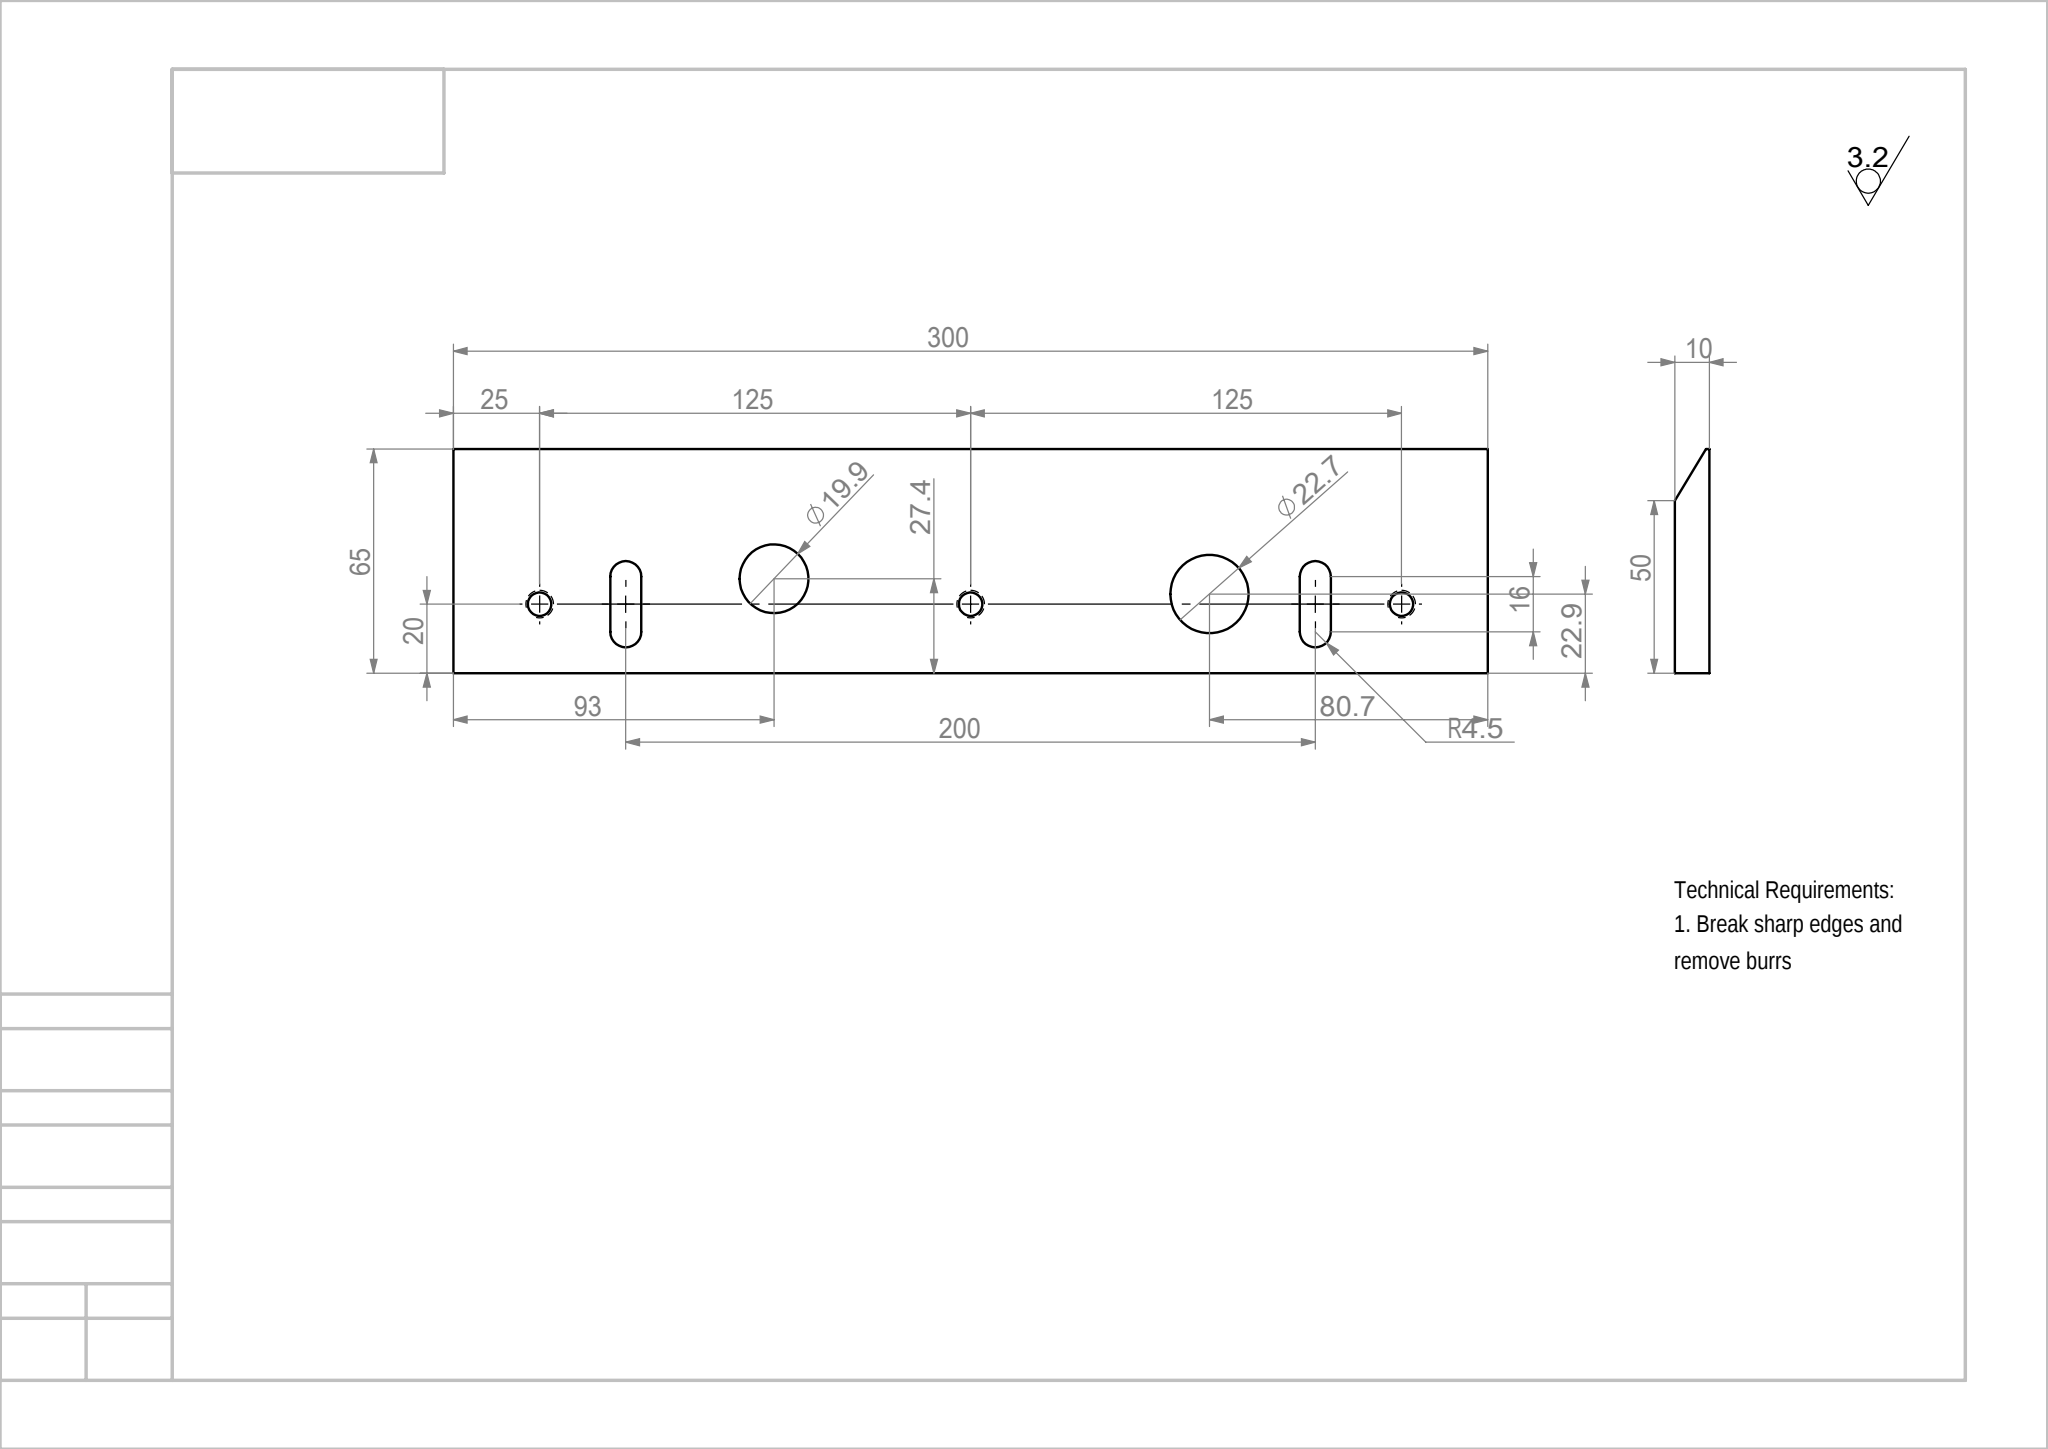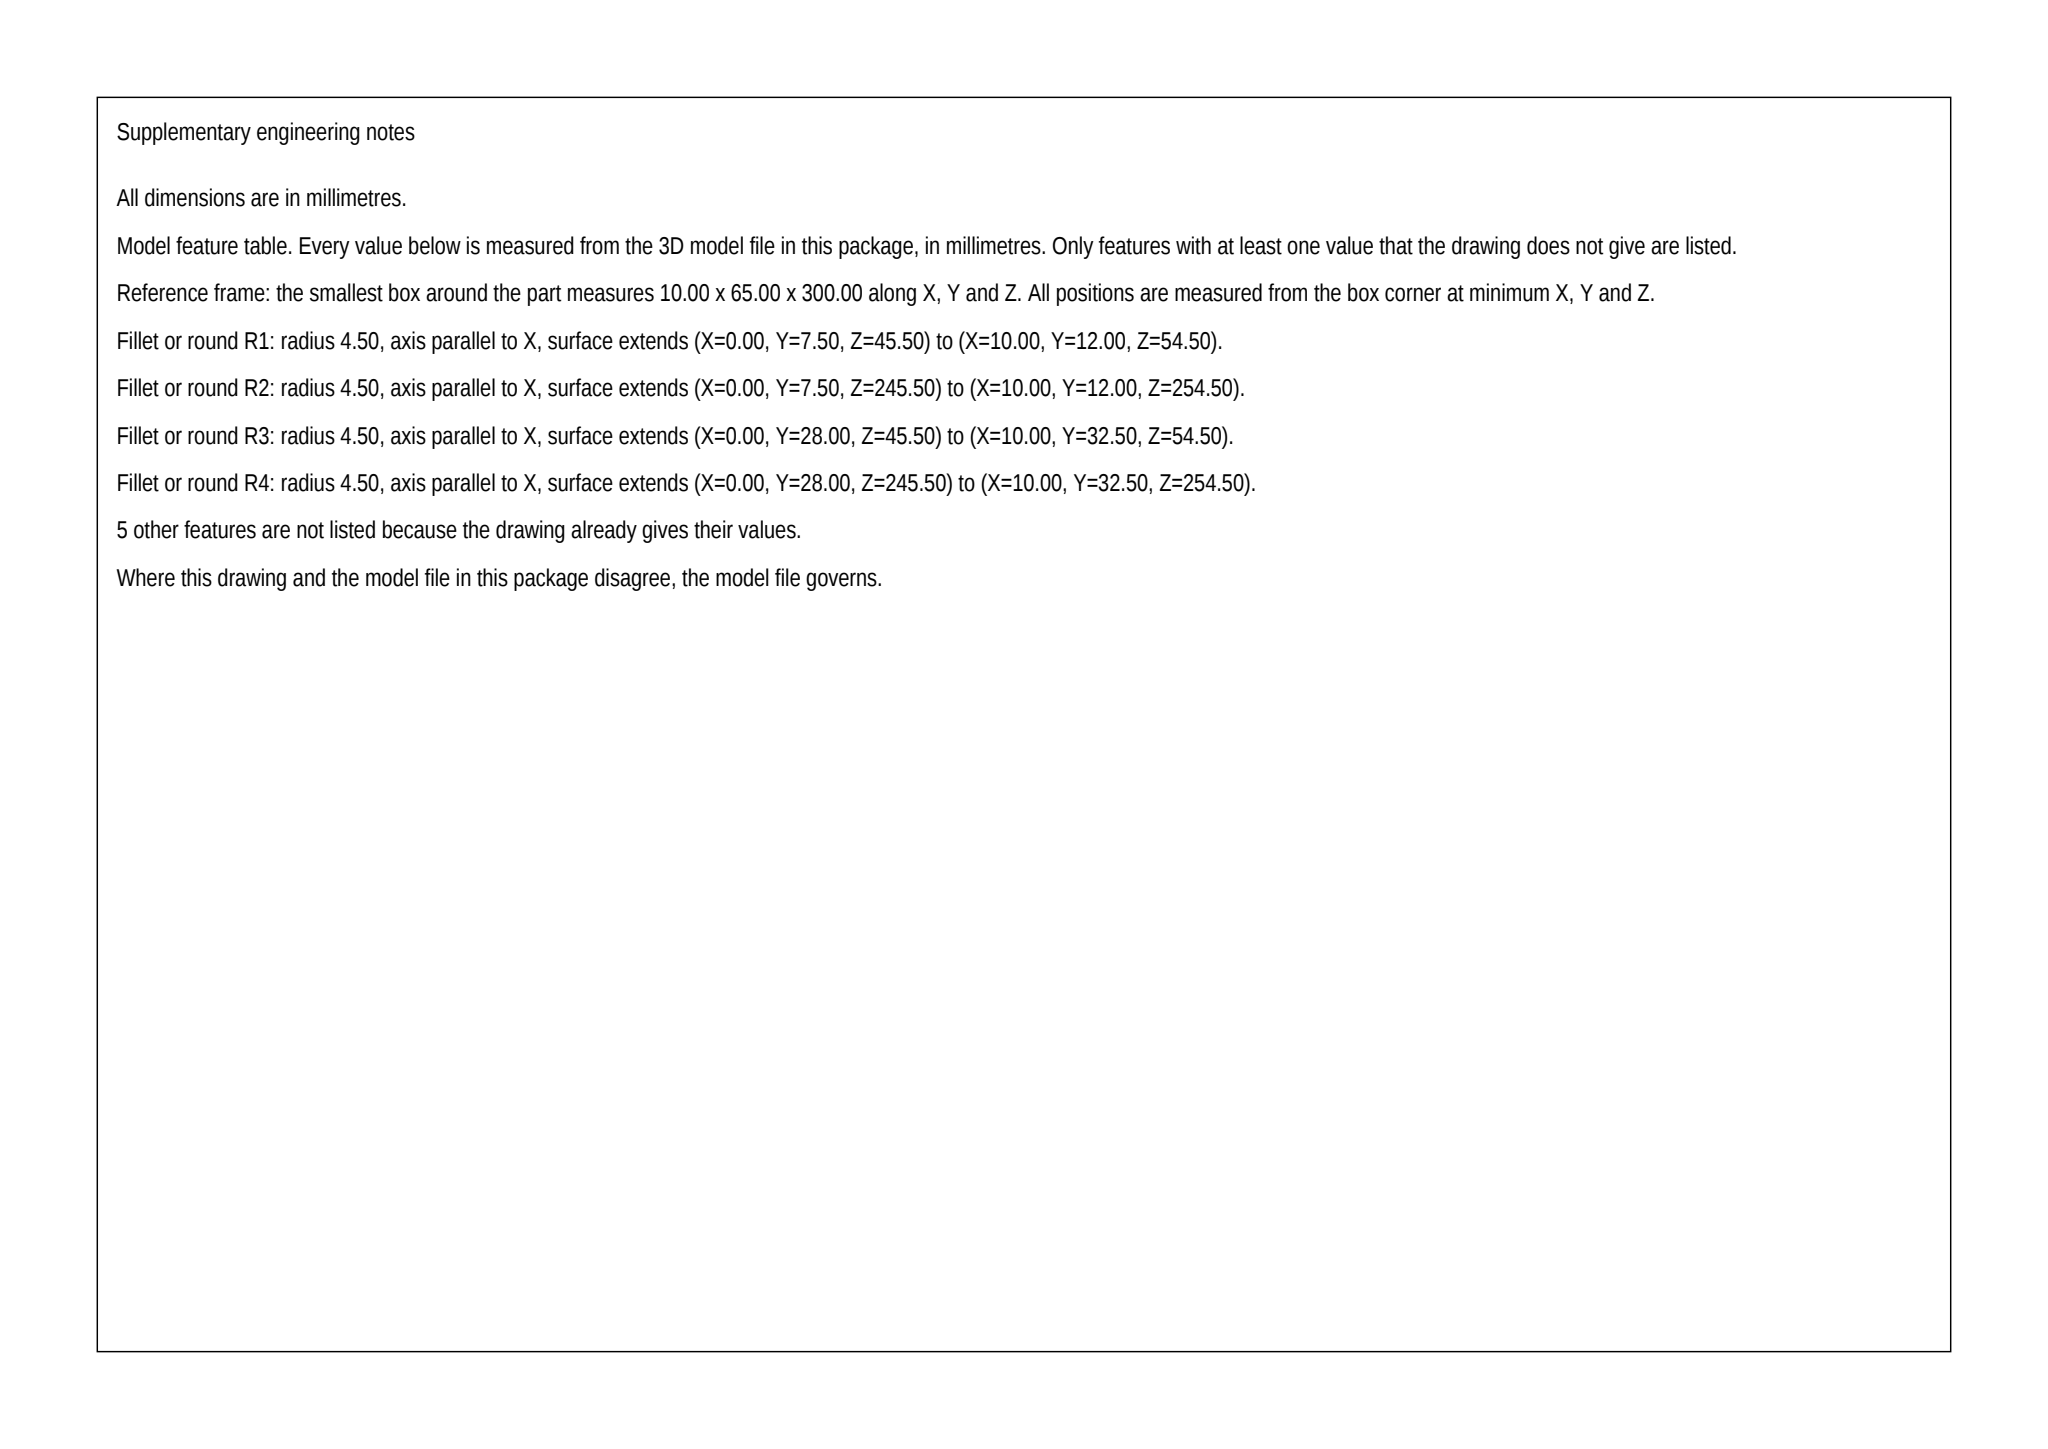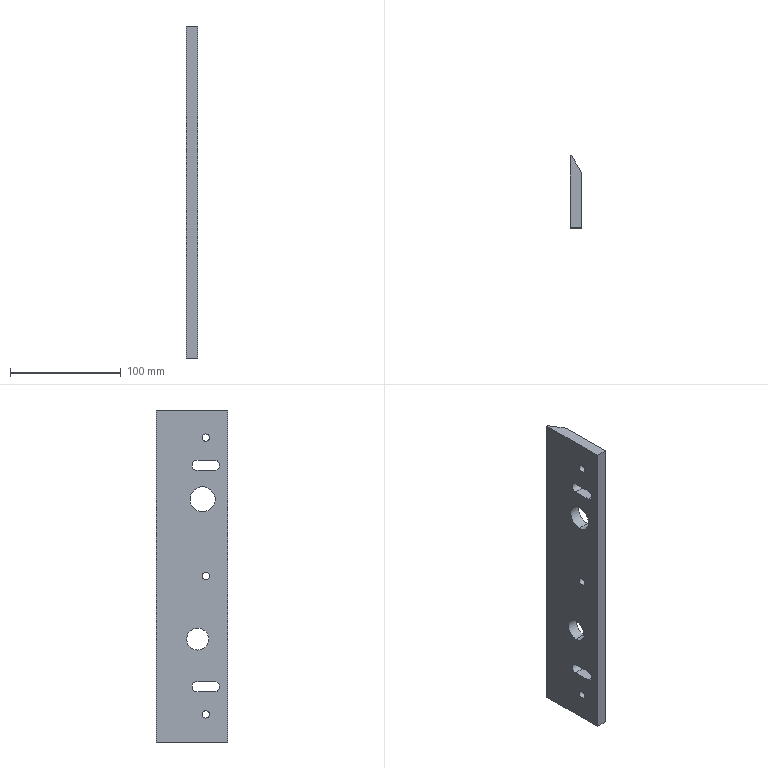Part | SolidWorks | mm | 1 solid | 25 faces | box 10 x 65 x 300 mm | volume 162340 mm3 | cylinder 14 | plane 11 | commonest cylinder face diameters 6.8 x6 9 x4 22.695 x2 19.94 x2
build123d program:
from build123d import *

# Parameters (mm, degrees)
BOSS_EXTRUDE1_DEPTH = 150
LPATTERN1_COUNT     = 3
LPATTERN1_PITCH     = 125
CUT_EXTRUDE1_DEPTH  = 10
SKETCH5_R           = 11.347
SKETCH5_R_2         = 9.97
CUT_EXTRUDE2_DEPTH  = 80


with BuildPart() as part:
    # Sketch1 → Boss-Extrude1 (new, symmetric)
    with BuildSketch(Plane.XY):
        Polygon((1, 65), (10, 50), (10, 0), (0, 0), (0, 65), align=None)
    extrude(amount=BOSS_EXTRUDE1_DEPTH, both=True)

    # Sketch3 → M8 Tapped Hole1 (revolve, cut)
    with BuildSketch(Plane(origin=(10, 20, 125), x_dir=(0, 0, -1), z_dir=(0, 1, 0))):
        Polygon((0, 0), (0, 41.793), (3.4, 39.75), (3.4, 0), align=None)
    m8_tapped_hole1 = revolve(axis=Axis((16.35, 20, 125), (-1, 0, 0)), mode=Mode.SUBTRACT)

    # LPattern1: M8 Tapped Hole1 ×3
    with Locations(*[(0, 0, -i * LPATTERN1_PITCH) for i in range(1, LPATTERN1_COUNT)]):
        add(m8_tapped_hole1, mode=Mode.SUBTRACT)

    # Sketch4 → Cut-Extrude1 (cut)
    with BuildSketch(Plane(origin=(10, 0, 0), x_dir=(0, 0, -1), z_dir=(1, 0, 0))):
        with BuildLine():
            Line((-104.5, 12), (-104.5, 28))
            ThreePointArc((-104.5, 28), (-100, 32.5), (-95.5, 28))
            Line((-95.5, 28), (-95.5, 12))
            ThreePointArc((-95.5, 12), (-100, 7.5), (-104.5, 12))
        make_face()
        with BuildLine():
            Line((104.5, 12), (104.5, 28))
            ThreePointArc((104.5, 28), (100, 32.5), (95.5, 28))
            Line((95.5, 28), (95.5, 12))
            ThreePointArc((95.5, 12), (100, 7.5), (104.5, 12))
        make_face()
    extrude(amount=-CUT_EXTRUDE1_DEPTH, mode=Mode.SUBTRACT)

    # Sketch5 → Cut-Extrude2 (cut)
    with BuildSketch(Plane(origin=(10, 0, 0), x_dir=(0, 0, -1), z_dir=(1, 0, 0))):
        with Locations((-69.297, 22.942)):
            Circle(SKETCH5_R)
        with Locations((57.008, 27.38)):
            Circle(SKETCH5_R_2)
    extrude(amount=-CUT_EXTRUDE2_DEPTH, mode=Mode.SUBTRACT)


solid = part.part
STEP:
#1=CARTESIAN_POINT('',(0.,22.942,80.644));
#2=VERTEX_POINT('',#1);
#3=CARTESIAN_POINT('',(0.,22.942,57.949));
#4=VERTEX_POINT('',#3);
#5=CARTESIAN_POINT('',(0.,22.942,69.297));
#6=DIRECTION('',(1.,0.,0.));
#7=DIRECTION('',(0.,0.,-1.));
#8=AXIS2_PLACEMENT_3D('',#5,#6,#7);
#9=CIRCLE('',#8,11.347);
#10=EDGE_CURVE('',#2,#4,#9,.T.);
#11=ORIENTED_EDGE('',*,*,#10,.F.);
#12=CARTESIAN_POINT('',(10.,22.942,80.644));
#13=VERTEX_POINT('',#12);
#14=CARTESIAN_POINT('',(-70.,22.942,80.644));
#15=DIRECTION('',(1.,0.,0.));
#16=VECTOR('',#15,1000.);
#17=LINE('',#14,#16);
#18=EDGE_CURVE('',#2,#13,#17,.T.);
#19=ORIENTED_EDGE('',*,*,#18,.T.);
#20=CARTESIAN_POINT('',(10.,22.942,57.949));
#21=VERTEX_POINT('',#20);
#22=CARTESIAN_POINT('',(10.,22.942,69.297));
#23=DIRECTION('',(1.,0.,0.));
#24=DIRECTION('',(0.,0.,-1.));
#25=AXIS2_PLACEMENT_3D('',#22,#23,#24);
#26=CIRCLE('',#25,11.347);
#27=EDGE_CURVE('',#13,#21,#26,.T.);
#28=ORIENTED_EDGE('',*,*,#27,.T.);
#29=CARTESIAN_POINT('',(-70.,22.942,57.949));
#30=DIRECTION('',(1.,0.,0.));
#31=VECTOR('',#30,1000.);
#32=LINE('',#29,#31);
#33=EDGE_CURVE('',#4,#21,#32,.T.);
#34=ORIENTED_EDGE('',*,*,#33,.F.);
#35=EDGE_LOOP('',(#11,#19,#28,#34));
#36=FACE_OUTER_BOUND('',#35,.T.);
#37=CARTESIAN_POINT('',(-70.,22.942,69.297));
#38=DIRECTION('',(1.,0.,0.));
#39=DIRECTION('',(0.,0.,-1.));
#40=AXIS2_PLACEMENT_3D('',#37,#38,#39);
#41=CYLINDRICAL_SURFACE('',#40,11.347);
#42=ADVANCED_FACE('',(#36),#41,.F.);
#43=CARTESIAN_POINT('',(0.,27.38,-47.038));
#44=VERTEX_POINT('',#43);
#45=CARTESIAN_POINT('',(0.,27.38,-66.978));
#46=VERTEX_POINT('',#45);
#47=CARTESIAN_POINT('',(0.,27.38,-57.008));
#48=DIRECTION('',(1.,0.,0.));
#49=DIRECTION('',(0.,0.,-1.));
#50=AXIS2_PLACEMENT_3D('',#47,#48,#49);
#51=CIRCLE('',#50,9.97);
#52=EDGE_CURVE('',#44,#46,#51,.T.);
#53=ORIENTED_EDGE('',*,*,#52,.F.);
#54=CARTESIAN_POINT('',(10.,27.38,-47.038));
#55=VERTEX_POINT('',#54);
#56=CARTESIAN_POINT('',(-70.,27.38,-47.038));
#57=DIRECTION('',(1.,0.,0.));
#58=VECTOR('',#57,1000.);
#59=LINE('',#56,#58);
#60=EDGE_CURVE('',#44,#55,#59,.T.);
#61=ORIENTED_EDGE('',*,*,#60,.T.);
#62=CARTESIAN_POINT('',(10.,27.38,-66.978));
#63=VERTEX_POINT('',#62);
#64=CARTESIAN_POINT('',(10.,27.38,-57.008));
#65=DIRECTION('',(1.,0.,0.));
#66=DIRECTION('',(0.,0.,-1.));
#67=AXIS2_PLACEMENT_3D('',#64,#65,#66);
#68=CIRCLE('',#67,9.97);
#69=EDGE_CURVE('',#55,#63,#68,.T.);
#70=ORIENTED_EDGE('',*,*,#69,.T.);
#71=CARTESIAN_POINT('',(-70.,27.38,-66.978));
#72=DIRECTION('',(1.,0.,0.));
#73=VECTOR('',#72,1000.);
#74=LINE('',#71,#73);
#75=EDGE_CURVE('',#46,#63,#74,.T.);
#76=ORIENTED_EDGE('',*,*,#75,.F.);
#77=EDGE_LOOP('',(#53,#61,#70,#76));
#78=FACE_OUTER_BOUND('',#77,.T.);
#79=CARTESIAN_POINT('',(-70.,27.38,-57.008));
#80=DIRECTION('',(1.,0.,0.));
#81=DIRECTION('',(0.,0.,-1.));
#82=AXIS2_PLACEMENT_3D('',#79,#80,#81);
#83=CYLINDRICAL_SURFACE('',#82,9.97);
#84=ADVANCED_FACE('',(#78),#83,.F.);
#85=CARTESIAN_POINT('',(0.,20.,-121.6));
#86=VERTEX_POINT('',#85);
#87=CARTESIAN_POINT('',(0.,20.,-128.4));
#88=VERTEX_POINT('',#87);
#89=CARTESIAN_POINT('',(0.,20.,-125.));
#90=DIRECTION('',(1.,0.,0.));
#91=DIRECTION('',(0.,0.,-1.));
#92=AXIS2_PLACEMENT_3D('',#89,#90,#91);
#93=CIRCLE('',#92,3.4);
#94=EDGE_CURVE('',#86,#88,#93,.T.);
#95=ORIENTED_EDGE('',*,*,#94,.F.);
#96=CARTESIAN_POINT('',(10.,20.,-121.6));
#97=VERTEX_POINT('',#96);
#98=CARTESIAN_POINT('',(10.,20.,-121.6));
#99=DIRECTION('',(1.,0.,0.));
#100=VECTOR('',#99,1000.);
#101=LINE('',#98,#100);
#102=EDGE_CURVE('',#86,#97,#101,.T.);
#103=ORIENTED_EDGE('',*,*,#102,.T.);
#104=CARTESIAN_POINT('',(10.,20.,-128.4));
#105=VERTEX_POINT('',#104);
#106=CARTESIAN_POINT('',(10.,20.,-125.));
#107=DIRECTION('',(1.,0.,0.));
#108=DIRECTION('',(0.,0.,-1.));
#109=AXIS2_PLACEMENT_3D('',#106,#107,#108);
#110=CIRCLE('',#109,3.4);
#111=EDGE_CURVE('',#97,#105,#110,.T.);
#112=ORIENTED_EDGE('',*,*,#111,.T.);
#113=CARTESIAN_POINT('',(10.,20.,-128.4));
#114=DIRECTION('',(1.,0.,0.));
#115=VECTOR('',#114,1000.);
#116=LINE('',#113,#115);
#117=EDGE_CURVE('',#88,#105,#116,.T.);
#118=ORIENTED_EDGE('',*,*,#117,.F.);
#119=EDGE_LOOP('',(#95,#103,#112,#118));
#120=FACE_OUTER_BOUND('',#119,.T.);
#121=CARTESIAN_POINT('',(10.,20.,-125.));
#122=DIRECTION('',(1.,0.,0.));
#123=DIRECTION('',(0.,0.,-1.));
#124=AXIS2_PLACEMENT_3D('',#121,#122,#123);
#125=CYLINDRICAL_SURFACE('',#124,3.4);
#126=ADVANCED_FACE('',(#120),#125,.F.);
#127=CARTESIAN_POINT('',(0.,20.,3.4));
#128=VERTEX_POINT('',#127);
#129=CARTESIAN_POINT('',(0.,20.,-3.4));
#130=VERTEX_POINT('',#129);
#131=CARTESIAN_POINT('',(0.,20.,0.));
#132=DIRECTION('',(1.,0.,0.));
#133=DIRECTION('',(0.,0.,-1.));
#134=AXIS2_PLACEMENT_3D('',#131,#132,#133);
#135=CIRCLE('',#134,3.4);
#136=EDGE_CURVE('',#128,#130,#135,.T.);
#137=ORIENTED_EDGE('',*,*,#136,.F.);
#138=CARTESIAN_POINT('',(10.,20.,3.4));
#139=VERTEX_POINT('',#138);
#140=CARTESIAN_POINT('',(10.,20.,3.4));
#141=DIRECTION('',(1.,0.,0.));
#142=VECTOR('',#141,1000.);
#143=LINE('',#140,#142);
#144=EDGE_CURVE('',#128,#139,#143,.T.);
#145=ORIENTED_EDGE('',*,*,#144,.T.);
#146=CARTESIAN_POINT('',(10.,20.,-3.4));
#147=VERTEX_POINT('',#146);
#148=CARTESIAN_POINT('',(10.,20.,0.));
#149=DIRECTION('',(1.,0.,0.));
#150=DIRECTION('',(0.,0.,-1.));
#151=AXIS2_PLACEMENT_3D('',#148,#149,#150);
#152=CIRCLE('',#151,3.4);
#153=EDGE_CURVE('',#139,#147,#152,.T.);
#154=ORIENTED_EDGE('',*,*,#153,.T.);
#155=CARTESIAN_POINT('',(10.,20.,-3.4));
#156=DIRECTION('',(1.,0.,0.));
#157=VECTOR('',#156,1000.);
#158=LINE('',#155,#157);
#159=EDGE_CURVE('',#130,#147,#158,.T.);
#160=ORIENTED_EDGE('',*,*,#159,.F.);
#161=EDGE_LOOP('',(#137,#145,#154,#160));
#162=FACE_OUTER_BOUND('',#161,.T.);
#163=CARTESIAN_POINT('',(10.,20.,0.));
#164=DIRECTION('',(1.,0.,0.));
#165=DIRECTION('',(0.,0.,-1.));
#166=AXIS2_PLACEMENT_3D('',#163,#164,#165);
#167=CYLINDRICAL_SURFACE('',#166,3.4);
#168=ADVANCED_FACE('',(#162),#167,.F.);
#169=CARTESIAN_POINT('',(0.,20.,128.4));
#170=VERTEX_POINT('',#169);
#171=CARTESIAN_POINT('',(0.,20.,121.6));
#172=VERTEX_POINT('',#171);
#173=CARTESIAN_POINT('',(0.,20.,125.));
#174=DIRECTION('',(1.,0.,0.));
#175=DIRECTION('',(0.,0.,-1.));
#176=AXIS2_PLACEMENT_3D('',#173,#174,#175);
#177=CIRCLE('',#176,3.4);
#178=EDGE_CURVE('',#170,#172,#177,.T.);
#179=ORIENTED_EDGE('',*,*,#178,.F.);
#180=CARTESIAN_POINT('',(10.,20.,128.4));
#181=VERTEX_POINT('',#180);
#182=CARTESIAN_POINT('',(10.,20.,128.4));
#183=DIRECTION('',(1.,0.,0.));
#184=VECTOR('',#183,1000.);
#185=LINE('',#182,#184);
#186=EDGE_CURVE('',#170,#181,#185,.T.);
#187=ORIENTED_EDGE('',*,*,#186,.T.);
#188=CARTESIAN_POINT('',(10.,20.,121.6));
#189=VERTEX_POINT('',#188);
#190=CARTESIAN_POINT('',(10.,20.,125.));
#191=DIRECTION('',(1.,0.,0.));
#192=DIRECTION('',(0.,0.,-1.));
#193=AXIS2_PLACEMENT_3D('',#190,#191,#192);
#194=CIRCLE('',#193,3.4);
#195=EDGE_CURVE('',#181,#189,#194,.T.);
#196=ORIENTED_EDGE('',*,*,#195,.T.);
#197=CARTESIAN_POINT('',(10.,20.,121.6));
#198=DIRECTION('',(1.,0.,0.));
#199=VECTOR('',#198,1000.);
#200=LINE('',#197,#199);
#201=EDGE_CURVE('',#172,#189,#200,.T.);
#202=ORIENTED_EDGE('',*,*,#201,.F.);
#203=EDGE_LOOP('',(#179,#187,#196,#202));
#204=FACE_OUTER_BOUND('',#203,.T.);
#205=CARTESIAN_POINT('',(10.,20.,125.));
#206=DIRECTION('',(1.,0.,0.));
#207=DIRECTION('',(0.,0.,-1.));
#208=AXIS2_PLACEMENT_3D('',#205,#206,#207);
#209=CYLINDRICAL_SURFACE('',#208,3.4);
#210=ADVANCED_FACE('',(#204),#209,.F.);
#211=CARTESIAN_POINT('',(0.,22.942,69.297));
#212=DIRECTION('',(1.,0.,0.));
#213=DIRECTION('',(0.,0.,-1.));
#214=AXIS2_PLACEMENT_3D('',#211,#212,#213);
#215=CIRCLE('',#214,11.347);
#216=EDGE_CURVE('',#4,#2,#215,.T.);
#217=ORIENTED_EDGE('',*,*,#216,.T.);
#218=ORIENTED_EDGE('',*,*,#10,.T.);
#219=EDGE_LOOP('',(#217,#218));
#220=FACE_BOUND('',#219,.T.);
#221=CARTESIAN_POINT('',(0.,27.38,-57.008));
#222=DIRECTION('',(1.,0.,0.));
#223=DIRECTION('',(0.,0.,-1.));
#224=AXIS2_PLACEMENT_3D('',#221,#222,#223);
#225=CIRCLE('',#224,9.97);
#226=EDGE_CURVE('',#46,#44,#225,.T.);
#227=ORIENTED_EDGE('',*,*,#226,.T.);
#228=ORIENTED_EDGE('',*,*,#52,.T.);
#229=EDGE_LOOP('',(#227,#228));
#230=FACE_BOUND('',#229,.T.);
#231=CARTESIAN_POINT('',(0.,28.,-95.5));
#232=VERTEX_POINT('',#231);
#233=CARTESIAN_POINT('',(0.,12.,-95.5));
#234=VERTEX_POINT('',#233);
#235=CARTESIAN_POINT('',(0.,12.,-95.5));
#236=DIRECTION('',(0.,-1.,0.));
#237=VECTOR('',#236,1000.);
#238=LINE('',#235,#237);
#239=EDGE_CURVE('',#232,#234,#238,.T.);
#240=ORIENTED_EDGE('',*,*,#239,.T.);
#241=CARTESIAN_POINT('',(0.,12.,-104.5));
#242=VERTEX_POINT('',#241);
#243=CARTESIAN_POINT('',(0.,12.,-100.));
#244=DIRECTION('',(1.,0.,0.));
#245=DIRECTION('',(0.,0.,1.));
#246=AXIS2_PLACEMENT_3D('',#243,#244,#245);
#247=CIRCLE('',#246,4.5);
#248=EDGE_CURVE('',#234,#242,#247,.T.);
#249=ORIENTED_EDGE('',*,*,#248,.T.);
#250=CARTESIAN_POINT('',(0.,28.,-104.5));
#251=VERTEX_POINT('',#250);
#252=CARTESIAN_POINT('',(0.,12.,-104.5));
#253=DIRECTION('',(0.,1.,0.));
#254=VECTOR('',#253,1000.);
#255=LINE('',#252,#254);
#256=EDGE_CURVE('',#242,#251,#255,.T.);
#257=ORIENTED_EDGE('',*,*,#256,.T.);
#258=CARTESIAN_POINT('',(0.,28.,-100.));
#259=DIRECTION('',(1.,0.,0.));
#260=DIRECTION('',(0.,0.,1.));
#261=AXIS2_PLACEMENT_3D('',#258,#259,#260);
#262=CIRCLE('',#261,4.5);
#263=EDGE_CURVE('',#251,#232,#262,.T.);
#264=ORIENTED_EDGE('',*,*,#263,.T.);
#265=EDGE_LOOP('',(#240,#249,#257,#264));
#266=FACE_BOUND('',#265,.T.);
#267=CARTESIAN_POINT('',(0.,28.,104.5));
#268=VERTEX_POINT('',#267);
#269=CARTESIAN_POINT('',(0.,12.,104.5));
#270=VERTEX_POINT('',#269);
#271=CARTESIAN_POINT('',(0.,12.,104.5));
#272=DIRECTION('',(0.,-1.,0.));
#273=VECTOR('',#272,1000.);
#274=LINE('',#271,#273);
#275=EDGE_CURVE('',#268,#270,#274,.T.);
#276=ORIENTED_EDGE('',*,*,#275,.T.);
#277=CARTESIAN_POINT('',(0.,12.,95.5));
#278=VERTEX_POINT('',#277);
#279=CARTESIAN_POINT('',(0.,12.,100.));
#280=DIRECTION('',(1.,0.,0.));
#281=DIRECTION('',(0.,0.,-1.));
#282=AXIS2_PLACEMENT_3D('',#279,#280,#281);
#283=CIRCLE('',#282,4.5);
#284=EDGE_CURVE('',#270,#278,#283,.T.);
#285=ORIENTED_EDGE('',*,*,#284,.T.);
#286=CARTESIAN_POINT('',(0.,28.,95.5));
#287=VERTEX_POINT('',#286);
#288=CARTESIAN_POINT('',(0.,12.,95.5));
#289=DIRECTION('',(0.,1.,0.));
#290=VECTOR('',#289,1000.);
#291=LINE('',#288,#290);
#292=EDGE_CURVE('',#278,#287,#291,.T.);
#293=ORIENTED_EDGE('',*,*,#292,.T.);
#294=CARTESIAN_POINT('',(0.,28.,100.));
#295=DIRECTION('',(1.,0.,0.));
#296=DIRECTION('',(0.,0.,-1.));
#297=AXIS2_PLACEMENT_3D('',#294,#295,#296);
#298=CIRCLE('',#297,4.5);
#299=EDGE_CURVE('',#287,#268,#298,.T.);
#300=ORIENTED_EDGE('',*,*,#299,.T.);
#301=EDGE_LOOP('',(#276,#285,#293,#300));
#302=FACE_BOUND('',#301,.T.);
#303=CARTESIAN_POINT('',(0.,20.,-125.));
#304=DIRECTION('',(1.,0.,0.));
#305=DIRECTION('',(0.,0.,-1.));
#306=AXIS2_PLACEMENT_3D('',#303,#304,#305);
#307=CIRCLE('',#306,3.4);
#308=EDGE_CURVE('',#88,#86,#307,.T.);
#309=ORIENTED_EDGE('',*,*,#308,.T.);
#310=ORIENTED_EDGE('',*,*,#94,.T.);
#311=EDGE_LOOP('',(#309,#310));
#312=FACE_BOUND('',#311,.T.);
#313=CARTESIAN_POINT('',(0.,20.,0.));
#314=DIRECTION('',(1.,0.,0.));
#315=DIRECTION('',(0.,0.,-1.));
#316=AXIS2_PLACEMENT_3D('',#313,#314,#315);
#317=CIRCLE('',#316,3.4);
#318=EDGE_CURVE('',#130,#128,#317,.T.);
#319=ORIENTED_EDGE('',*,*,#318,.T.);
#320=ORIENTED_EDGE('',*,*,#136,.T.);
#321=EDGE_LOOP('',(#319,#320));
#322=FACE_BOUND('',#321,.T.);
#323=CARTESIAN_POINT('',(0.,20.,125.));
#324=DIRECTION('',(1.,0.,0.));
#325=DIRECTION('',(0.,0.,-1.));
#326=AXIS2_PLACEMENT_3D('',#323,#324,#325);
#327=CIRCLE('',#326,3.4);
#328=EDGE_CURVE('',#172,#170,#327,.T.);
#329=ORIENTED_EDGE('',*,*,#328,.T.);
#330=ORIENTED_EDGE('',*,*,#178,.T.);
#331=EDGE_LOOP('',(#329,#330));
#332=FACE_BOUND('',#331,.T.);
#333=CARTESIAN_POINT('',(0.,65.,-150.));
#334=VERTEX_POINT('',#333);
#335=CARTESIAN_POINT('',(0.,0.,-150.));
#336=VERTEX_POINT('',#335);
#337=CARTESIAN_POINT('',(0.,0.,-150.));
#338=DIRECTION('',(0.,-1.,0.));
#339=VECTOR('',#338,1000.);
#340=LINE('',#337,#339);
#341=EDGE_CURVE('',#334,#336,#340,.T.);
#342=ORIENTED_EDGE('',*,*,#341,.T.);
#343=CARTESIAN_POINT('',(0.,0.,150.));
#344=VERTEX_POINT('',#343);
#345=CARTESIAN_POINT('',(0.,0.,150.));
#346=DIRECTION('',(0.,0.,-1.));
#347=VECTOR('',#346,1000.);
#348=LINE('',#345,#347);
#349=EDGE_CURVE('',#344,#336,#348,.T.);
#350=ORIENTED_EDGE('',*,*,#349,.F.);
#351=CARTESIAN_POINT('',(0.,65.,150.));
#352=VERTEX_POINT('',#351);
#353=CARTESIAN_POINT('',(0.,0.,150.));
#354=DIRECTION('',(0.,-1.,0.));
#355=VECTOR('',#354,1000.);
#356=LINE('',#353,#355);
#357=EDGE_CURVE('',#352,#344,#356,.T.);
#358=ORIENTED_EDGE('',*,*,#357,.F.);
#359=CARTESIAN_POINT('',(0.,65.,150.));
#360=DIRECTION('',(0.,0.,-1.));
#361=VECTOR('',#360,1000.);
#362=LINE('',#359,#361);
#363=EDGE_CURVE('',#352,#334,#362,.T.);
#364=ORIENTED_EDGE('',*,*,#363,.T.);
#365=EDGE_LOOP('',(#342,#350,#358,#364));
#366=FACE_OUTER_BOUND('',#365,.T.);
#367=CARTESIAN_POINT('',(0.,0.,150.));
#368=DIRECTION('',(1.,0.,0.));
#369=DIRECTION('',(0.,0.,-1.));
#370=AXIS2_PLACEMENT_3D('',#367,#368,#369);
#371=PLANE('',#370);
#372=ADVANCED_FACE('',(#220,#230,#266,#302,#312,#322,#332,#366),#371,.F.);
#373=CARTESIAN_POINT('',(10.,0.,-150.));
#374=VERTEX_POINT('',#373);
#375=CARTESIAN_POINT('',(0.,0.,-150.));
#376=DIRECTION('',(1.,0.,0.));
#377=VECTOR('',#376,1000.);
#378=LINE('',#375,#377);
#379=EDGE_CURVE('',#336,#374,#378,.T.);
#380=ORIENTED_EDGE('',*,*,#379,.T.);
#381=CARTESIAN_POINT('',(10.,0.,150.));
#382=VERTEX_POINT('',#381);
#383=CARTESIAN_POINT('',(10.,0.,150.));
#384=DIRECTION('',(0.,0.,-1.));
#385=VECTOR('',#384,1000.);
#386=LINE('',#383,#385);
#387=EDGE_CURVE('',#382,#374,#386,.T.);
#388=ORIENTED_EDGE('',*,*,#387,.F.);
#389=CARTESIAN_POINT('',(0.,0.,150.));
#390=DIRECTION('',(1.,0.,0.));
#391=VECTOR('',#390,1000.);
#392=LINE('',#389,#391);
#393=EDGE_CURVE('',#344,#382,#392,.T.);
#394=ORIENTED_EDGE('',*,*,#393,.F.);
#395=ORIENTED_EDGE('',*,*,#349,.T.);
#396=EDGE_LOOP('',(#380,#388,#394,#395));
#397=FACE_OUTER_BOUND('',#396,.T.);
#398=CARTESIAN_POINT('',(0.,0.,150.));
#399=DIRECTION('',(0.,1.,0.));
#400=DIRECTION('',(0.,0.,1.));
#401=AXIS2_PLACEMENT_3D('',#398,#399,#400);
#402=PLANE('',#401);
#403=ADVANCED_FACE('',(#397),#402,.F.);
#404=CARTESIAN_POINT('',(10.,22.942,69.297));
#405=DIRECTION('',(1.,0.,0.));
#406=DIRECTION('',(0.,0.,-1.));
#407=AXIS2_PLACEMENT_3D('',#404,#405,#406);
#408=CIRCLE('',#407,11.347);
#409=EDGE_CURVE('',#21,#13,#408,.T.);
#410=ORIENTED_EDGE('',*,*,#409,.F.);
#411=ORIENTED_EDGE('',*,*,#27,.F.);
#412=EDGE_LOOP('',(#410,#411));
#413=FACE_BOUND('',#412,.T.);
#414=CARTESIAN_POINT('',(10.,27.38,-57.008));
#415=DIRECTION('',(1.,0.,0.));
#416=DIRECTION('',(0.,0.,-1.));
#417=AXIS2_PLACEMENT_3D('',#414,#415,#416);
#418=CIRCLE('',#417,9.97);
#419=EDGE_CURVE('',#63,#55,#418,.T.);
#420=ORIENTED_EDGE('',*,*,#419,.F.);
#421=ORIENTED_EDGE('',*,*,#69,.F.);
#422=EDGE_LOOP('',(#420,#421));
#423=FACE_BOUND('',#422,.T.);
#424=CARTESIAN_POINT('',(10.,12.,-104.5));
#425=VERTEX_POINT('',#424);
#426=CARTESIAN_POINT('',(10.,28.,-104.5));
#427=VERTEX_POINT('',#426);
#428=CARTESIAN_POINT('',(10.,12.,-104.5));
#429=DIRECTION('',(0.,1.,0.));
#430=VECTOR('',#429,1000.);
#431=LINE('',#428,#430);
#432=EDGE_CURVE('',#425,#427,#431,.T.);
#433=ORIENTED_EDGE('',*,*,#432,.F.);
#434=CARTESIAN_POINT('',(10.,12.,-95.5));
#435=VERTEX_POINT('',#434);
#436=CARTESIAN_POINT('',(10.,12.,-100.));
#437=DIRECTION('',(1.,0.,0.));
#438=DIRECTION('',(0.,0.,1.));
#439=AXIS2_PLACEMENT_3D('',#436,#437,#438);
#440=CIRCLE('',#439,4.5);
#441=EDGE_CURVE('',#435,#425,#440,.T.);
#442=ORIENTED_EDGE('',*,*,#441,.F.);
#443=CARTESIAN_POINT('',(10.,28.,-95.5));
#444=VERTEX_POINT('',#443);
#445=CARTESIAN_POINT('',(10.,12.,-95.5));
#446=DIRECTION('',(0.,-1.,0.));
#447=VECTOR('',#446,1000.);
#448=LINE('',#445,#447);
#449=EDGE_CURVE('',#444,#435,#448,.T.);
#450=ORIENTED_EDGE('',*,*,#449,.F.);
#451=CARTESIAN_POINT('',(10.,28.,-100.));
#452=DIRECTION('',(1.,0.,0.));
#453=DIRECTION('',(0.,0.,1.));
#454=AXIS2_PLACEMENT_3D('',#451,#452,#453);
#455=CIRCLE('',#454,4.5);
#456=EDGE_CURVE('',#427,#444,#455,.T.);
#457=ORIENTED_EDGE('',*,*,#456,.F.);
#458=EDGE_LOOP('',(#433,#442,#450,#457));
#459=FACE_BOUND('',#458,.T.);
#460=CARTESIAN_POINT('',(10.,12.,95.5));
#461=VERTEX_POINT('',#460);
#462=CARTESIAN_POINT('',(10.,28.,95.5));
#463=VERTEX_POINT('',#462);
#464=CARTESIAN_POINT('',(10.,12.,95.5));
#465=DIRECTION('',(0.,1.,0.));
#466=VECTOR('',#465,1000.);
#467=LINE('',#464,#466);
#468=EDGE_CURVE('',#461,#463,#467,.T.);
#469=ORIENTED_EDGE('',*,*,#468,.F.);
#470=CARTESIAN_POINT('',(10.,12.,104.5));
#471=VERTEX_POINT('',#470);
#472=CARTESIAN_POINT('',(10.,12.,100.));
#473=DIRECTION('',(1.,0.,0.));
#474=DIRECTION('',(0.,0.,-1.));
#475=AXIS2_PLACEMENT_3D('',#472,#473,#474);
#476=CIRCLE('',#475,4.5);
#477=EDGE_CURVE('',#471,#461,#476,.T.);
#478=ORIENTED_EDGE('',*,*,#477,.F.);
#479=CARTESIAN_POINT('',(10.,28.,104.5));
#480=VERTEX_POINT('',#479);
#481=CARTESIAN_POINT('',(10.,12.,104.5));
#482=DIRECTION('',(0.,-1.,0.));
#483=VECTOR('',#482,1000.);
#484=LINE('',#481,#483);
#485=EDGE_CURVE('',#480,#471,#484,.T.);
#486=ORIENTED_EDGE('',*,*,#485,.F.);
#487=CARTESIAN_POINT('',(10.,28.,100.));
#488=DIRECTION('',(1.,0.,0.));
#489=DIRECTION('',(0.,0.,-1.));
#490=AXIS2_PLACEMENT_3D('',#487,#488,#489);
#491=CIRCLE('',#490,4.5);
#492=EDGE_CURVE('',#463,#480,#491,.T.);
#493=ORIENTED_EDGE('',*,*,#492,.F.);
#494=EDGE_LOOP('',(#469,#478,#486,#493));
#495=FACE_BOUND('',#494,.T.);
#496=CARTESIAN_POINT('',(10.,20.,-125.));
#497=DIRECTION('',(1.,0.,0.));
#498=DIRECTION('',(0.,0.,-1.));
#499=AXIS2_PLACEMENT_3D('',#496,#497,#498);
#500=CIRCLE('',#499,3.4);
#501=EDGE_CURVE('',#105,#97,#500,.T.);
#502=ORIENTED_EDGE('',*,*,#501,.F.);
#503=ORIENTED_EDGE('',*,*,#111,.F.);
#504=EDGE_LOOP('',(#502,#503));
#505=FACE_BOUND('',#504,.T.);
#506=CARTESIAN_POINT('',(10.,20.,0.));
#507=DIRECTION('',(1.,0.,0.));
#508=DIRECTION('',(0.,0.,-1.));
#509=AXIS2_PLACEMENT_3D('',#506,#507,#508);
#510=CIRCLE('',#509,3.4);
#511=EDGE_CURVE('',#147,#139,#510,.T.);
#512=ORIENTED_EDGE('',*,*,#511,.F.);
#513=ORIENTED_EDGE('',*,*,#153,.F.);
#514=EDGE_LOOP('',(#512,#513));
#515=FACE_BOUND('',#514,.T.);
#516=CARTESIAN_POINT('',(10.,20.,125.));
#517=DIRECTION('',(1.,0.,0.));
#518=DIRECTION('',(0.,0.,-1.));
#519=AXIS2_PLACEMENT_3D('',#516,#517,#518);
#520=CIRCLE('',#519,3.4);
#521=EDGE_CURVE('',#189,#181,#520,.T.);
#522=ORIENTED_EDGE('',*,*,#521,.F.);
#523=ORIENTED_EDGE('',*,*,#195,.F.);
#524=EDGE_LOOP('',(#522,#523));
#525=FACE_BOUND('',#524,.T.);
#526=CARTESIAN_POINT('',(10.,50.,-150.));
#527=VERTEX_POINT('',#526);
#528=CARTESIAN_POINT('',(10.,0.,-150.));
#529=DIRECTION('',(0.,1.,0.));
#530=VECTOR('',#529,1000.);
#531=LINE('',#528,#530);
#532=EDGE_CURVE('',#374,#527,#531,.T.);
#533=ORIENTED_EDGE('',*,*,#532,.T.);
#534=CARTESIAN_POINT('',(10.,50.,150.));
#535=VERTEX_POINT('',#534);
#536=CARTESIAN_POINT('',(10.,50.,150.));
#537=DIRECTION('',(0.,0.,-1.));
#538=VECTOR('',#537,1000.);
#539=LINE('',#536,#538);
#540=EDGE_CURVE('',#535,#527,#539,.T.);
#541=ORIENTED_EDGE('',*,*,#540,.F.);
#542=CARTESIAN_POINT('',(10.,0.,150.));
#543=DIRECTION('',(0.,1.,0.));
#544=VECTOR('',#543,1000.);
#545=LINE('',#542,#544);
#546=EDGE_CURVE('',#382,#535,#545,.T.);
#547=ORIENTED_EDGE('',*,*,#546,.F.);
#548=ORIENTED_EDGE('',*,*,#387,.T.);
#549=EDGE_LOOP('',(#533,#541,#547,#548));
#550=FACE_OUTER_BOUND('',#549,.T.);
#551=CARTESIAN_POINT('',(10.,0.,150.));
#552=DIRECTION('',(-1.,0.,0.));
#553=DIRECTION('',(0.,0.,1.));
#554=AXIS2_PLACEMENT_3D('',#551,#552,#553);
#555=PLANE('',#554);
#556=ADVANCED_FACE('',(#413,#423,#459,#495,#505,#515,#525,#550),#555,.F.);
#557=CARTESIAN_POINT('',(1.,65.,-150.));
#558=VERTEX_POINT('',#557);
#559=CARTESIAN_POINT('',(1.,65.,-150.));
#560=DIRECTION('',(-0.5145,0.8575,0.));
#561=VECTOR('',#560,1000.);
#562=LINE('',#559,#561);
#563=EDGE_CURVE('',#527,#558,#562,.T.);
#564=ORIENTED_EDGE('',*,*,#563,.T.);
#565=CARTESIAN_POINT('',(1.,65.,150.));
#566=VERTEX_POINT('',#565);
#567=CARTESIAN_POINT('',(1.,65.,150.));
#568=DIRECTION('',(0.,0.,-1.));
#569=VECTOR('',#568,1000.);
#570=LINE('',#567,#569);
#571=EDGE_CURVE('',#566,#558,#570,.T.);
#572=ORIENTED_EDGE('',*,*,#571,.F.);
#573=CARTESIAN_POINT('',(1.,65.,150.));
#574=DIRECTION('',(-0.5145,0.8575,0.));
#575=VECTOR('',#574,1000.);
#576=LINE('',#573,#575);
#577=EDGE_CURVE('',#535,#566,#576,.T.);
#578=ORIENTED_EDGE('',*,*,#577,.F.);
#579=ORIENTED_EDGE('',*,*,#540,.T.);
#580=EDGE_LOOP('',(#564,#572,#578,#579));
#581=FACE_OUTER_BOUND('',#580,.T.);
#582=CARTESIAN_POINT('',(1.,65.,150.));
#583=DIRECTION('',(-0.8575,-0.5145,0.));
#584=DIRECTION('',(0.5145,-0.8575,0.));
#585=AXIS2_PLACEMENT_3D('',#582,#583,#584);
#586=PLANE('',#585);
#587=ADVANCED_FACE('',(#581),#586,.F.);
#588=CARTESIAN_POINT('',(0.,65.,-150.));
#589=DIRECTION('',(-1.,0.,0.));
#590=VECTOR('',#589,1000.);
#591=LINE('',#588,#590);
#592=EDGE_CURVE('',#558,#334,#591,.T.);
#593=ORIENTED_EDGE('',*,*,#592,.T.);
#594=ORIENTED_EDGE('',*,*,#363,.F.);
#595=CARTESIAN_POINT('',(0.,65.,150.));
#596=DIRECTION('',(-1.,0.,0.));
#597=VECTOR('',#596,1000.);
#598=LINE('',#595,#597);
#599=EDGE_CURVE('',#566,#352,#598,.T.);
#600=ORIENTED_EDGE('',*,*,#599,.F.);
#601=ORIENTED_EDGE('',*,*,#571,.T.);
#602=EDGE_LOOP('',(#593,#594,#600,#601));
#603=FACE_OUTER_BOUND('',#602,.T.);
#604=CARTESIAN_POINT('',(0.,65.,150.));
#605=DIRECTION('',(0.,-1.,0.));
#606=DIRECTION('',(0.,0.,-1.));
#607=AXIS2_PLACEMENT_3D('',#604,#605,#606);
#608=PLANE('',#607);
#609=ADVANCED_FACE('',(#603),#608,.F.);
#610=ORIENTED_EDGE('',*,*,#357,.T.);
#611=ORIENTED_EDGE('',*,*,#393,.T.);
#612=ORIENTED_EDGE('',*,*,#546,.T.);
#613=ORIENTED_EDGE('',*,*,#577,.T.);
#614=ORIENTED_EDGE('',*,*,#599,.T.);
#615=EDGE_LOOP('',(#610,#611,#612,#613,#614));
#616=FACE_OUTER_BOUND('',#615,.T.);
#617=CARTESIAN_POINT('',(0.,65.,150.));
#618=DIRECTION('',(0.,0.,-1.));
#619=DIRECTION('',(-1.,0.,0.));
#620=AXIS2_PLACEMENT_3D('',#617,#618,#619);
#621=PLANE('',#620);
#622=ADVANCED_FACE('',(#616),#621,.F.);
#623=ORIENTED_EDGE('',*,*,#341,.F.);
#624=ORIENTED_EDGE('',*,*,#592,.F.);
#625=ORIENTED_EDGE('',*,*,#563,.F.);
#626=ORIENTED_EDGE('',*,*,#532,.F.);
#627=ORIENTED_EDGE('',*,*,#379,.F.);
#628=EDGE_LOOP('',(#623,#624,#625,#626,#627));
#629=FACE_OUTER_BOUND('',#628,.T.);
#630=CARTESIAN_POINT('',(0.,65.,-150.));
#631=DIRECTION('',(0.,0.,-1.));
#632=DIRECTION('',(-1.,0.,0.));
#633=AXIS2_PLACEMENT_3D('',#630,#631,#632);
#634=PLANE('',#633);
#635=ADVANCED_FACE('',(#629),#634,.T.);
#636=ORIENTED_EDGE('',*,*,#186,.F.);
#637=ORIENTED_EDGE('',*,*,#328,.F.);
#638=ORIENTED_EDGE('',*,*,#201,.T.);
#639=ORIENTED_EDGE('',*,*,#521,.T.);
#640=EDGE_LOOP('',(#636,#637,#638,#639));
#641=FACE_OUTER_BOUND('',#640,.T.);
#642=CARTESIAN_POINT('',(10.,20.,125.));
#643=DIRECTION('',(1.,0.,0.));
#644=DIRECTION('',(0.,0.,-1.));
#645=AXIS2_PLACEMENT_3D('',#642,#643,#644);
#646=CYLINDRICAL_SURFACE('',#645,3.4);
#647=ADVANCED_FACE('',(#641),#646,.F.);
#648=ORIENTED_EDGE('',*,*,#144,.F.);
#649=ORIENTED_EDGE('',*,*,#318,.F.);
#650=ORIENTED_EDGE('',*,*,#159,.T.);
#651=ORIENTED_EDGE('',*,*,#511,.T.);
#652=EDGE_LOOP('',(#648,#649,#650,#651));
#653=FACE_OUTER_BOUND('',#652,.T.);
#654=CARTESIAN_POINT('',(10.,20.,0.));
#655=DIRECTION('',(1.,0.,0.));
#656=DIRECTION('',(0.,0.,-1.));
#657=AXIS2_PLACEMENT_3D('',#654,#655,#656);
#658=CYLINDRICAL_SURFACE('',#657,3.4);
#659=ADVANCED_FACE('',(#653),#658,.F.);
#660=ORIENTED_EDGE('',*,*,#102,.F.);
#661=ORIENTED_EDGE('',*,*,#308,.F.);
#662=ORIENTED_EDGE('',*,*,#117,.T.);
#663=ORIENTED_EDGE('',*,*,#501,.T.);
#664=EDGE_LOOP('',(#660,#661,#662,#663));
#665=FACE_OUTER_BOUND('',#664,.T.);
#666=CARTESIAN_POINT('',(10.,20.,-125.));
#667=DIRECTION('',(1.,0.,0.));
#668=DIRECTION('',(0.,0.,-1.));
#669=AXIS2_PLACEMENT_3D('',#666,#667,#668);
#670=CYLINDRICAL_SURFACE('',#669,3.4);
#671=ADVANCED_FACE('',(#665),#670,.F.);
#672=ORIENTED_EDGE('',*,*,#477,.T.);
#673=CARTESIAN_POINT('',(0.,12.,95.5));
#674=DIRECTION('',(1.,0.,0.));
#675=VECTOR('',#674,1000.);
#676=LINE('',#673,#675);
#677=EDGE_CURVE('',#278,#461,#676,.T.);
#678=ORIENTED_EDGE('',*,*,#677,.F.);
#679=ORIENTED_EDGE('',*,*,#284,.F.);
#680=CARTESIAN_POINT('',(0.,12.,104.5));
#681=DIRECTION('',(1.,0.,0.));
#682=VECTOR('',#681,1000.);
#683=LINE('',#680,#682);
#684=EDGE_CURVE('',#270,#471,#683,.T.);
#685=ORIENTED_EDGE('',*,*,#684,.T.);
#686=EDGE_LOOP('',(#672,#678,#679,#685));
#687=FACE_OUTER_BOUND('',#686,.T.);
#688=CARTESIAN_POINT('',(0.,12.,100.));
#689=DIRECTION('',(1.,0.,0.));
#690=DIRECTION('',(0.,0.,-1.));
#691=AXIS2_PLACEMENT_3D('',#688,#689,#690);
#692=CYLINDRICAL_SURFACE('',#691,4.5);
#693=ADVANCED_FACE('',(#687),#692,.F.);
#694=ORIENTED_EDGE('',*,*,#485,.T.);
#695=ORIENTED_EDGE('',*,*,#684,.F.);
#696=ORIENTED_EDGE('',*,*,#275,.F.);
#697=CARTESIAN_POINT('',(0.,28.,104.5));
#698=DIRECTION('',(1.,0.,0.));
#699=VECTOR('',#698,1000.);
#700=LINE('',#697,#699);
#701=EDGE_CURVE('',#268,#480,#700,.T.);
#702=ORIENTED_EDGE('',*,*,#701,.T.);
#703=EDGE_LOOP('',(#694,#695,#696,#702));
#704=FACE_OUTER_BOUND('',#703,.T.);
#705=CARTESIAN_POINT('',(0.,12.,104.5));
#706=DIRECTION('',(0.,0.,1.));
#707=DIRECTION('',(1.,0.,0.));
#708=AXIS2_PLACEMENT_3D('',#705,#706,#707);
#709=PLANE('',#708);
#710=ADVANCED_FACE('',(#704),#709,.F.);
#711=ORIENTED_EDGE('',*,*,#492,.T.);
#712=ORIENTED_EDGE('',*,*,#701,.F.);
#713=ORIENTED_EDGE('',*,*,#299,.F.);
#714=CARTESIAN_POINT('',(0.,28.,95.5));
#715=DIRECTION('',(1.,0.,0.));
#716=VECTOR('',#715,1000.);
#717=LINE('',#714,#716);
#718=EDGE_CURVE('',#287,#463,#717,.T.);
#719=ORIENTED_EDGE('',*,*,#718,.T.);
#720=EDGE_LOOP('',(#711,#712,#713,#719));
#721=FACE_OUTER_BOUND('',#720,.T.);
#722=CARTESIAN_POINT('',(0.,28.,100.));
#723=DIRECTION('',(1.,0.,0.));
#724=DIRECTION('',(0.,0.,-1.));
#725=AXIS2_PLACEMENT_3D('',#722,#723,#724);
#726=CYLINDRICAL_SURFACE('',#725,4.5);
#727=ADVANCED_FACE('',(#721),#726,.F.);
#728=ORIENTED_EDGE('',*,*,#468,.T.);
#729=ORIENTED_EDGE('',*,*,#718,.F.);
#730=ORIENTED_EDGE('',*,*,#292,.F.);
#731=ORIENTED_EDGE('',*,*,#677,.T.);
#732=EDGE_LOOP('',(#728,#729,#730,#731));
#733=FACE_OUTER_BOUND('',#732,.T.);
#734=CARTESIAN_POINT('',(0.,12.,95.5));
#735=DIRECTION('',(0.,0.,-1.));
#736=DIRECTION('',(-1.,0.,0.));
#737=AXIS2_PLACEMENT_3D('',#734,#735,#736);
#738=PLANE('',#737);
#739=ADVANCED_FACE('',(#733),#738,.F.);
#740=ORIENTED_EDGE('',*,*,#441,.T.);
#741=CARTESIAN_POINT('',(0.,12.,-104.5));
#742=DIRECTION('',(1.,0.,0.));
#743=VECTOR('',#742,1000.);
#744=LINE('',#741,#743);
#745=EDGE_CURVE('',#242,#425,#744,.T.);
#746=ORIENTED_EDGE('',*,*,#745,.F.);
#747=ORIENTED_EDGE('',*,*,#248,.F.);
#748=CARTESIAN_POINT('',(0.,12.,-95.5));
#749=DIRECTION('',(1.,0.,0.));
#750=VECTOR('',#749,1000.);
#751=LINE('',#748,#750);
#752=EDGE_CURVE('',#234,#435,#751,.T.);
#753=ORIENTED_EDGE('',*,*,#752,.T.);
#754=EDGE_LOOP('',(#740,#746,#747,#753));
#755=FACE_OUTER_BOUND('',#754,.T.);
#756=CARTESIAN_POINT('',(0.,12.,-100.));
#757=DIRECTION('',(1.,0.,0.));
#758=DIRECTION('',(0.,0.,-1.));
#759=AXIS2_PLACEMENT_3D('',#756,#757,#758);
#760=CYLINDRICAL_SURFACE('',#759,4.5);
#761=ADVANCED_FACE('',(#755),#760,.F.);
#762=ORIENTED_EDGE('',*,*,#449,.T.);
#763=ORIENTED_EDGE('',*,*,#752,.F.);
#764=ORIENTED_EDGE('',*,*,#239,.F.);
#765=CARTESIAN_POINT('',(0.,28.,-95.5));
#766=DIRECTION('',(1.,0.,0.));
#767=VECTOR('',#766,1000.);
#768=LINE('',#765,#767);
#769=EDGE_CURVE('',#232,#444,#768,.T.);
#770=ORIENTED_EDGE('',*,*,#769,.T.);
#771=EDGE_LOOP('',(#762,#763,#764,#770));
#772=FACE_OUTER_BOUND('',#771,.T.);
#773=CARTESIAN_POINT('',(0.,12.,-95.5));
#774=DIRECTION('',(0.,0.,1.));
#775=DIRECTION('',(1.,0.,0.));
#776=AXIS2_PLACEMENT_3D('',#773,#774,#775);
#777=PLANE('',#776);
#778=ADVANCED_FACE('',(#772),#777,.F.);
#779=ORIENTED_EDGE('',*,*,#456,.T.);
#780=ORIENTED_EDGE('',*,*,#769,.F.);
#781=ORIENTED_EDGE('',*,*,#263,.F.);
#782=CARTESIAN_POINT('',(0.,28.,-104.5));
#783=DIRECTION('',(1.,0.,0.));
#784=VECTOR('',#783,1000.);
#785=LINE('',#782,#784);
#786=EDGE_CURVE('',#251,#427,#785,.T.);
#787=ORIENTED_EDGE('',*,*,#786,.T.);
#788=EDGE_LOOP('',(#779,#780,#781,#787));
#789=FACE_OUTER_BOUND('',#788,.T.);
#790=CARTESIAN_POINT('',(0.,28.,-100.));
#791=DIRECTION('',(1.,0.,0.));
#792=DIRECTION('',(0.,0.,-1.));
#793=AXIS2_PLACEMENT_3D('',#790,#791,#792);
#794=CYLINDRICAL_SURFACE('',#793,4.5);
#795=ADVANCED_FACE('',(#789),#794,.F.);
#796=ORIENTED_EDGE('',*,*,#432,.T.);
#797=ORIENTED_EDGE('',*,*,#786,.F.);
#798=ORIENTED_EDGE('',*,*,#256,.F.);
#799=ORIENTED_EDGE('',*,*,#745,.T.);
#800=EDGE_LOOP('',(#796,#797,#798,#799));
#801=FACE_OUTER_BOUND('',#800,.T.);
#802=CARTESIAN_POINT('',(0.,12.,-104.5));
#803=DIRECTION('',(0.,0.,-1.));
#804=DIRECTION('',(-1.,0.,0.));
#805=AXIS2_PLACEMENT_3D('',#802,#803,#804);
#806=PLANE('',#805);
#807=ADVANCED_FACE('',(#801),#806,.F.);
#808=ORIENTED_EDGE('',*,*,#60,.F.);
#809=ORIENTED_EDGE('',*,*,#226,.F.);
#810=ORIENTED_EDGE('',*,*,#75,.T.);
#811=ORIENTED_EDGE('',*,*,#419,.T.);
#812=EDGE_LOOP('',(#808,#809,#810,#811));
#813=FACE_OUTER_BOUND('',#812,.T.);
#814=CARTESIAN_POINT('',(-70.,27.38,-57.008));
#815=DIRECTION('',(1.,0.,0.));
#816=DIRECTION('',(0.,0.,-1.));
#817=AXIS2_PLACEMENT_3D('',#814,#815,#816);
#818=CYLINDRICAL_SURFACE('',#817,9.97);
#819=ADVANCED_FACE('',(#813),#818,.F.);
#820=ORIENTED_EDGE('',*,*,#18,.F.);
#821=ORIENTED_EDGE('',*,*,#216,.F.);
#822=ORIENTED_EDGE('',*,*,#33,.T.);
#823=ORIENTED_EDGE('',*,*,#409,.T.);
#824=EDGE_LOOP('',(#820,#821,#822,#823));
#825=FACE_OUTER_BOUND('',#824,.T.);
#826=CARTESIAN_POINT('',(-70.,22.942,69.297));
#827=DIRECTION('',(1.,0.,0.));
#828=DIRECTION('',(0.,0.,-1.));
#829=AXIS2_PLACEMENT_3D('',#826,#827,#828);
#830=CYLINDRICAL_SURFACE('',#829,11.347);
#831=ADVANCED_FACE('',(#825),#830,.F.);
#832=CLOSED_SHELL('',(#42,#84,#126,#168,#210,#372,#403,#556,#587,#609,#622,#635,#647,#659,#671,#693,#710,#727,#739,#761,#778,#795,#807,#819,#831));
#833=MANIFOLD_SOLID_BREP('',#832);
#834=CARTESIAN_POINT('',(0.,0.,0.));
#835=DIRECTION('',(0.,0.,1.));
#836=DIRECTION('',(1.,0.,0.));
#837=AXIS2_PLACEMENT_3D('',#834,#835,#836);
#838=(LENGTH_UNIT()NAMED_UNIT(*)SI_UNIT(.MILLI.,.METRE.));
#839=UNCERTAINTY_MEASURE_WITH_UNIT(LENGTH_MEASURE(0.00001),#838,'','');
#840=(NAMED_UNIT(*)PLANE_ANGLE_UNIT()SI_UNIT($,.RADIAN.));
#841=(NAMED_UNIT(*)SI_UNIT($,.STERADIAN.)SOLID_ANGLE_UNIT());
#842=(GEOMETRIC_REPRESENTATION_CONTEXT(3)GLOBAL_UNCERTAINTY_ASSIGNED_CONTEXT((#839))GLOBAL_UNIT_ASSIGNED_CONTEXT((#838,#840,#841))REPRESENTATION_CONTEXT('',''));
#843=ADVANCED_BREP_SHAPE_REPRESENTATION('',(#833,#837),#842);